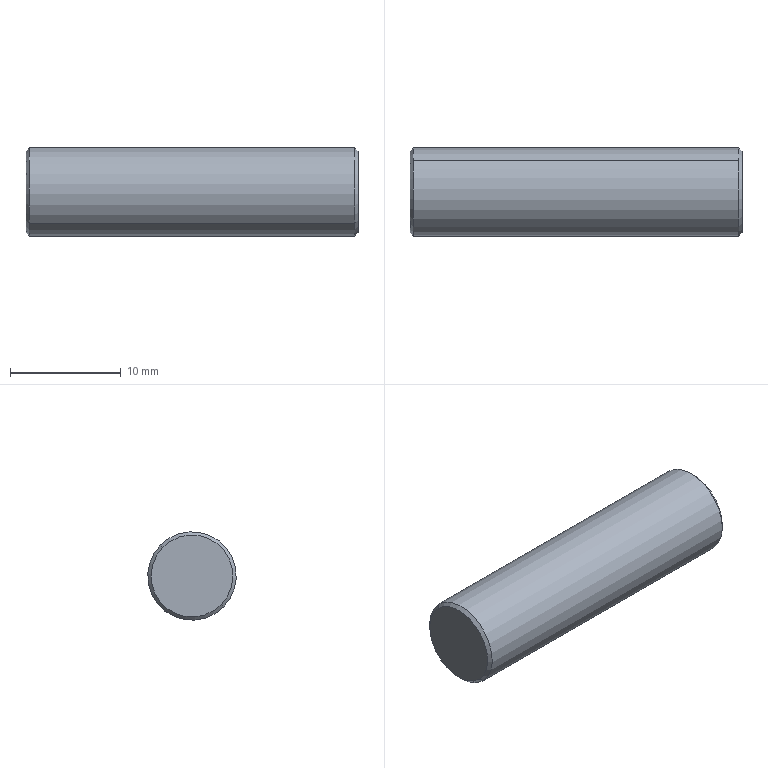Component | SolidWorks | HingeAssembly-1_Pin-1 | 1 solid | 8 faces | box 30 x 8 x 8 mm | volume 1506 mm3 | cone 4 | cylinder 2 | plane 2 | commonest cylinder face diameters 8 x2
build123d program:
from build123d import *

# Parameters (mm, degrees)
SKETCH1_R           = 4
BOSS_EXTRUDE1_DEPTH = 30
CHAMFER1_SIZE       = 0.3


with BuildPart() as part:
    # Sketch1 → Boss-Extrude1 (new body)
    with BuildSketch(Plane.XY):
        Circle(SKETCH1_R)
    extrude(amount=BOSS_EXTRUDE1_DEPTH)

    # Chamfer1
    chamfer1_edges = [part.edges().sort_by_distance(p)[0] for p in [
        (-4, 0, 0),
        (-4, 0, 30),
    ]]
    chamfer(chamfer1_edges, length=CHAMFER1_SIZE)


solid = part.part

# Placed as in the assembly
solid = solid.moved(Location((-749.848, -185.605, 361), (0, 90, 0)))
STEP:
#1=COLOUR_RGB('',0.7922,0.8196,0.9333);
#2=FILL_AREA_STYLE_COLOUR('',#1);
#3=FILL_AREA_STYLE('',(#2));
#4=SURFACE_STYLE_FILL_AREA(#3);
#5=SURFACE_SIDE_STYLE('',(#4));
#6=SURFACE_STYLE_USAGE(.BOTH.,#5);
#7=PRESENTATION_STYLE_ASSIGNMENT((#6));
#8=CARTESIAN_POINT('',(-28.34,-7.204,14.315));
#9=VERTEX_POINT('',#8);
#10=CARTESIAN_POINT('',(-28.34,-7.411,14.11));
#11=VERTEX_POINT('',#10);
#12=CARTESIAN_POINT('',(-28.34,-7.307,14.213));
#13=DIRECTION('',(1.,0.,-0.));
#14=DIRECTION('',(0.,0.7118,0.7023));
#15=AXIS2_PLACEMENT_3D('',#12,#13,#14);
#16=CIRCLE('',#15,0.1457);
#17=EDGE_CURVE('',#9,#11,#16,.T.);
#18=ORIENTED_EDGE('',*,*,#17,.F.);
#19=CARTESIAN_POINT('',(-28.352,-7.195,14.323));
#20=VERTEX_POINT('',#19);
#21=CARTESIAN_POINT('',(-28.34,-7.204,14.315));
#22=DIRECTION('',(-0.7071,0.5033,0.4966));
#23=VECTOR('',#22,39.37);
#24=LINE('',#21,#23);
#25=EDGE_CURVE('',#9,#20,#24,.T.);
#26=ORIENTED_EDGE('',*,*,#25,.T.);
#27=CARTESIAN_POINT('',(-28.352,-7.419,14.102));
#28=VERTEX_POINT('',#27);
#29=CARTESIAN_POINT('',(-28.352,-7.307,14.213));
#30=DIRECTION('',(-1.,-0.,0.));
#31=DIRECTION('',(0.,0.7118,0.7023));
#32=AXIS2_PLACEMENT_3D('',#29,#30,#31);
#33=CIRCLE('',#32,0.1575);
#34=EDGE_CURVE('',#28,#20,#33,.T.);
#35=ORIENTED_EDGE('',*,*,#34,.F.);
#36=CARTESIAN_POINT('',(-28.34,-7.411,14.11));
#37=DIRECTION('',(-0.7071,-0.5033,-0.4966));
#38=VECTOR('',#37,39.37);
#39=LINE('',#36,#38);
#40=EDGE_CURVE('',#11,#28,#39,.T.);
#41=ORIENTED_EDGE('',*,*,#40,.F.);
#42=EDGE_LOOP('',(#18,#26,#35,#41));
#43=FACE_OUTER_BOUND('',#42,.T.);
#44=CARTESIAN_POINT('',(-28.34,-7.307,14.213));
#45=DIRECTION('',(-1.,-0.,0.));
#46=DIRECTION('',(0.,-0.7118,-0.7023));
#47=AXIS2_PLACEMENT_3D('',#44,#45,#46);
#48=CONICAL_SURFACE('',#47,0.1457,0.7854);
#49=ADVANCED_FACE('',(#43),#48,.T.);
#50=CARTESIAN_POINT('',(-29.522,-7.411,14.11));
#51=VERTEX_POINT('',#50);
#52=CARTESIAN_POINT('',(-29.522,-7.204,14.315));
#53=VERTEX_POINT('',#52);
#54=CARTESIAN_POINT('',(-29.522,-7.307,14.213));
#55=DIRECTION('',(-1.,-0.,0.));
#56=DIRECTION('',(0.,0.7118,0.7023));
#57=AXIS2_PLACEMENT_3D('',#54,#55,#56);
#58=CIRCLE('',#57,0.1457);
#59=EDGE_CURVE('',#51,#53,#58,.T.);
#60=ORIENTED_EDGE('',*,*,#59,.F.);
#61=CARTESIAN_POINT('',(-29.51,-7.419,14.102));
#62=VERTEX_POINT('',#61);
#63=CARTESIAN_POINT('',(-29.51,-7.419,14.102));
#64=DIRECTION('',(0.7071,-0.5033,-0.4966));
#65=VECTOR('',#64,39.37);
#66=LINE('',#63,#65);
#67=EDGE_CURVE('',#51,#62,#66,.T.);
#68=ORIENTED_EDGE('',*,*,#67,.T.);
#69=CARTESIAN_POINT('',(-29.51,-7.195,14.323));
#70=VERTEX_POINT('',#69);
#71=CARTESIAN_POINT('',(-29.51,-7.307,14.213));
#72=DIRECTION('',(1.,0.,-0.));
#73=DIRECTION('',(0.,0.7118,0.7023));
#74=AXIS2_PLACEMENT_3D('',#71,#72,#73);
#75=CIRCLE('',#74,0.1575);
#76=EDGE_CURVE('',#70,#62,#75,.T.);
#77=ORIENTED_EDGE('',*,*,#76,.F.);
#78=CARTESIAN_POINT('',(-29.51,-7.195,14.323));
#79=DIRECTION('',(0.7071,0.5033,0.4966));
#80=VECTOR('',#79,39.37);
#81=LINE('',#78,#80);
#82=EDGE_CURVE('',#53,#70,#81,.T.);
#83=ORIENTED_EDGE('',*,*,#82,.F.);
#84=EDGE_LOOP('',(#60,#68,#77,#83));
#85=FACE_OUTER_BOUND('',#84,.T.);
#86=CARTESIAN_POINT('',(-29.51,-7.307,14.213));
#87=DIRECTION('',(1.,0.,-0.));
#88=DIRECTION('',(0.,0.7118,0.7023));
#89=AXIS2_PLACEMENT_3D('',#86,#87,#88);
#90=CONICAL_SURFACE('',#89,0.1575,0.7854);
#91=ADVANCED_FACE('',(#85),#90,.T.);
#92=ORIENTED_EDGE('',*,*,#34,.T.);
#93=CARTESIAN_POINT('',(-28.34,-7.195,14.323));
#94=DIRECTION('',(-1.,-0.,0.));
#95=VECTOR('',#94,39.37);
#96=LINE('',#93,#95);
#97=EDGE_CURVE('',#20,#70,#96,.T.);
#98=ORIENTED_EDGE('',*,*,#97,.T.);
#99=ORIENTED_EDGE('',*,*,#76,.T.);
#100=CARTESIAN_POINT('',(-28.34,-7.419,14.102));
#101=DIRECTION('',(-1.,-0.,0.));
#102=VECTOR('',#101,39.37);
#103=LINE('',#100,#102);
#104=EDGE_CURVE('',#28,#62,#103,.T.);
#105=ORIENTED_EDGE('',*,*,#104,.F.);
#106=EDGE_LOOP('',(#92,#98,#99,#105));
#107=FACE_OUTER_BOUND('',#106,.T.);
#108=CARTESIAN_POINT('',(-28.34,-7.307,14.213));
#109=DIRECTION('',(-1.,-0.,0.));
#110=DIRECTION('',(0.,-0.7118,-0.7023));
#111=AXIS2_PLACEMENT_3D('',#108,#109,#110);
#112=CYLINDRICAL_SURFACE('',#111,0.1575);
#113=ADVANCED_FACE('',(#107),#112,.T.);
#114=ORIENTED_EDGE('',*,*,#97,.F.);
#115=CARTESIAN_POINT('',(-28.352,-7.307,14.213));
#116=DIRECTION('',(-1.,-0.,0.));
#117=DIRECTION('',(0.,0.7118,0.7023));
#118=AXIS2_PLACEMENT_3D('',#115,#116,#117);
#119=CIRCLE('',#118,0.1575);
#120=EDGE_CURVE('',#20,#28,#119,.T.);
#121=ORIENTED_EDGE('',*,*,#120,.T.);
#122=ORIENTED_EDGE('',*,*,#104,.T.);
#123=CARTESIAN_POINT('',(-29.51,-7.307,14.213));
#124=DIRECTION('',(1.,0.,-0.));
#125=DIRECTION('',(0.,0.7118,0.7023));
#126=AXIS2_PLACEMENT_3D('',#123,#124,#125);
#127=CIRCLE('',#126,0.1575);
#128=EDGE_CURVE('',#62,#70,#127,.T.);
#129=ORIENTED_EDGE('',*,*,#128,.T.);
#130=EDGE_LOOP('',(#114,#121,#122,#129));
#131=FACE_OUTER_BOUND('',#130,.T.);
#132=CARTESIAN_POINT('',(-28.34,-7.307,14.213));
#133=DIRECTION('',(-1.,-0.,0.));
#134=DIRECTION('',(0.,-0.7118,-0.7023));
#135=AXIS2_PLACEMENT_3D('',#132,#133,#134);
#136=CYLINDRICAL_SURFACE('',#135,0.1575);
#137=ADVANCED_FACE('',(#131),#136,.T.);
#138=CARTESIAN_POINT('',(-28.34,-7.307,14.213));
#139=DIRECTION('',(1.,0.,-0.));
#140=DIRECTION('',(0.,0.7118,0.7023));
#141=AXIS2_PLACEMENT_3D('',#138,#139,#140);
#142=CIRCLE('',#141,0.1457);
#143=EDGE_CURVE('',#11,#9,#142,.T.);
#144=ORIENTED_EDGE('',*,*,#143,.T.);
#145=ORIENTED_EDGE('',*,*,#17,.T.);
#146=EDGE_LOOP('',(#144,#145));
#147=FACE_OUTER_BOUND('',#146,.T.);
#148=CARTESIAN_POINT('',(-28.34,-7.307,14.213));
#149=DIRECTION('',(1.,0.,-0.));
#150=DIRECTION('',(-0.,0.7118,0.7023));
#151=AXIS2_PLACEMENT_3D('',#148,#149,#150);
#152=PLANE('',#151);
#153=ADVANCED_FACE('',(#147),#152,.T.);
#154=CARTESIAN_POINT('',(-29.522,-7.307,14.213));
#155=DIRECTION('',(-1.,-0.,0.));
#156=DIRECTION('',(0.,0.7118,0.7023));
#157=AXIS2_PLACEMENT_3D('',#154,#155,#156);
#158=CIRCLE('',#157,0.1457);
#159=EDGE_CURVE('',#53,#51,#158,.T.);
#160=ORIENTED_EDGE('',*,*,#159,.T.);
#161=ORIENTED_EDGE('',*,*,#59,.T.);
#162=EDGE_LOOP('',(#160,#161));
#163=FACE_OUTER_BOUND('',#162,.T.);
#164=CARTESIAN_POINT('',(-29.522,-7.307,14.213));
#165=DIRECTION('',(1.,0.,-0.));
#166=DIRECTION('',(-0.,0.7118,0.7023));
#167=AXIS2_PLACEMENT_3D('',#164,#165,#166);
#168=PLANE('',#167);
#169=ADVANCED_FACE('',(#163),#168,.F.);
#170=ORIENTED_EDGE('',*,*,#67,.F.);
#171=ORIENTED_EDGE('',*,*,#159,.F.);
#172=ORIENTED_EDGE('',*,*,#82,.T.);
#173=ORIENTED_EDGE('',*,*,#128,.F.);
#174=EDGE_LOOP('',(#170,#171,#172,#173));
#175=FACE_OUTER_BOUND('',#174,.T.);
#176=CARTESIAN_POINT('',(-29.51,-7.307,14.213));
#177=DIRECTION('',(1.,0.,-0.));
#178=DIRECTION('',(0.,0.7118,0.7023));
#179=AXIS2_PLACEMENT_3D('',#176,#177,#178);
#180=CONICAL_SURFACE('',#179,0.1575,0.7854);
#181=ADVANCED_FACE('',(#175),#180,.T.);
#182=ORIENTED_EDGE('',*,*,#25,.F.);
#183=ORIENTED_EDGE('',*,*,#143,.F.);
#184=ORIENTED_EDGE('',*,*,#40,.T.);
#185=ORIENTED_EDGE('',*,*,#120,.F.);
#186=EDGE_LOOP('',(#182,#183,#184,#185));
#187=FACE_OUTER_BOUND('',#186,.T.);
#188=CARTESIAN_POINT('',(-28.34,-7.307,14.213));
#189=DIRECTION('',(-1.,-0.,0.));
#190=DIRECTION('',(0.,-0.7118,-0.7023));
#191=AXIS2_PLACEMENT_3D('',#188,#189,#190);
#192=CONICAL_SURFACE('',#191,0.1457,0.7854);
#193=ADVANCED_FACE('',(#187),#192,.T.);
#194=CLOSED_SHELL('',(#49,#91,#113,#137,#153,#169,#181,#193));
#195=MANIFOLD_SOLID_BREP('',#194);
#196=STYLED_ITEM('',(#7),#195);
#197=PRESENTATION_LAYER_ASSIGNMENT('','',(#196));
#198=(LENGTH_UNIT()NAMED_UNIT(*)SI_UNIT($,.METRE.));
#199=LENGTH_MEASURE_WITH_UNIT(LENGTH_MEASURE(0.0254),#198);
#200=DIMENSIONAL_EXPONENTS(1.,0.,0.,0.,0.,0.,0.);
#201=(CONVERSION_BASED_UNIT('',#199)LENGTH_UNIT()NAMED_UNIT(#200));
#202=UNCERTAINTY_MEASURE_WITH_UNIT(LENGTH_MEASURE(0.00001),#201,'','');
#203=(NAMED_UNIT(*)PLANE_ANGLE_UNIT()SI_UNIT($,.RADIAN.));
#204=(NAMED_UNIT(*)SI_UNIT($,.STERADIAN.)SOLID_ANGLE_UNIT());
#205=(GEOMETRIC_REPRESENTATION_CONTEXT(3)GLOBAL_UNCERTAINTY_ASSIGNED_CONTEXT((#202))GLOBAL_UNIT_ASSIGNED_CONTEXT((#201,#203,#204))REPRESENTATION_CONTEXT('',''));
#206=MECHANICAL_DESIGN_GEOMETRIC_PRESENTATION_REPRESENTATION('',(#196),#205);
#207=CARTESIAN_POINT('',(0.,0.,0.));
#208=DIRECTION('',(0.,0.,1.));
#209=DIRECTION('',(1.,0.,0.));
#210=AXIS2_PLACEMENT_3D('',#207,#208,#209);
#211=(LENGTH_UNIT()NAMED_UNIT(*)SI_UNIT($,.METRE.));
#212=LENGTH_MEASURE_WITH_UNIT(LENGTH_MEASURE(0.0254),#211);
#213=DIMENSIONAL_EXPONENTS(1.,0.,0.,0.,0.,0.,0.);
#214=(CONVERSION_BASED_UNIT('',#212)LENGTH_UNIT()NAMED_UNIT(#213));
#215=UNCERTAINTY_MEASURE_WITH_UNIT(LENGTH_MEASURE(0.00001),#214,'','');
#216=(NAMED_UNIT(*)PLANE_ANGLE_UNIT()SI_UNIT($,.RADIAN.));
#217=(NAMED_UNIT(*)SI_UNIT($,.STERADIAN.)SOLID_ANGLE_UNIT());
#218=(GEOMETRIC_REPRESENTATION_CONTEXT(3)GLOBAL_UNCERTAINTY_ASSIGNED_CONTEXT((#215))GLOBAL_UNIT_ASSIGNED_CONTEXT((#214,#216,#217))REPRESENTATION_CONTEXT('',''));
#219=ADVANCED_BREP_SHAPE_REPRESENTATION('',(#195,#210),#218);